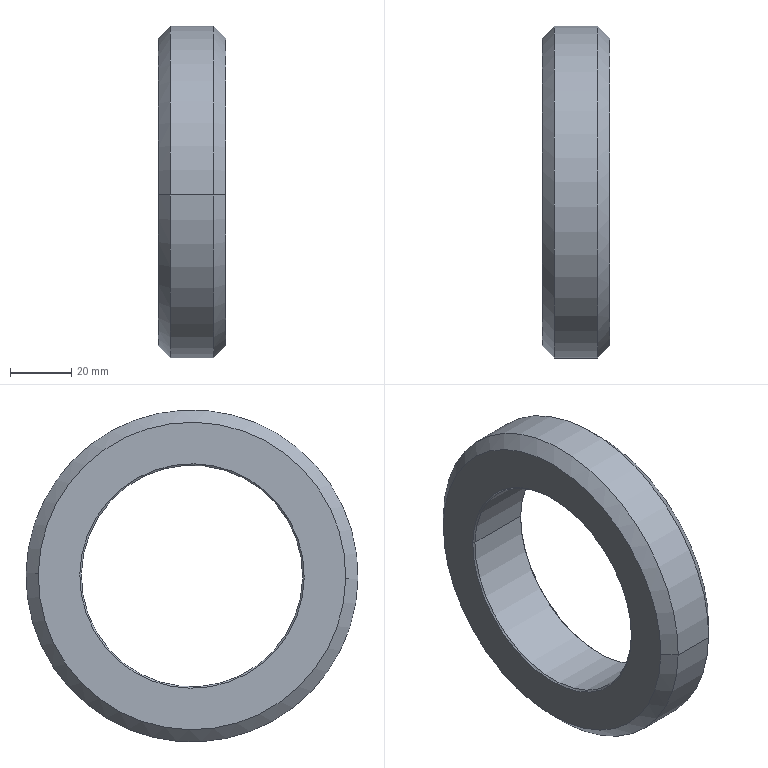Component | SolidWorks | 216InnerTubeAssembly-1_HangingRing-1 | 1 solid | 14 faces | box 22 x 108 x 108 mm | volume 106615 mm3 | cone 8 | cylinder 4 | plane 2 | commonest cylinder face diameters 108 x2 72 x2 | material Alloy Steel
build123d program:
from build123d import *


with BuildPart() as part:
    # Model → Revolve1 (revolve)
    with BuildSketch(Plane.XY):
        Polygon((-0.3448, 49.996), (-0.3448, 36.496), (-0.8448, 35.996), (-21.845, 35.996), (-22.345, 36.496), (-22.345, 49.996), (-18.345, 53.996), (-4.345, 53.996), align=None)
    revolve(axis=Axis((-0.1895, -0.00351, 0), (-1, 0, 0)))


solid = part.part

# Placed as in the assembly
solid = solid.moved(Location((650.924, 0.00351, 0), (0, 0, 0)))
STEP:
#1=CARTESIAN_POINT('',(24.905,2.126,0.03817));
#2=VERTEX_POINT('',#1);
#3=CARTESIAN_POINT('',(24.905,-2.126,-0.03817));
#4=VERTEX_POINT('',#3);
#5=CARTESIAN_POINT('',(24.905,-0.,0.));
#6=DIRECTION('',(1.,0.,0.));
#7=DIRECTION('',(0.,0.9998,0.01796));
#8=AXIS2_PLACEMENT_3D('',#5,#6,#7);
#9=CIRCLE('',#8,2.126);
#10=EDGE_CURVE('',#2,#4,#9,.T.);
#11=ORIENTED_EDGE('',*,*,#10,.T.);
#12=CARTESIAN_POINT('',(25.456,-2.126,-0.03817));
#13=VERTEX_POINT('',#12);
#14=CARTESIAN_POINT('',(25.619,-2.126,-0.03817));
#15=DIRECTION('',(1.,0.,0.));
#16=VECTOR('',#15,39.37);
#17=LINE('',#14,#16);
#18=EDGE_CURVE('',#4,#13,#17,.T.);
#19=ORIENTED_EDGE('',*,*,#18,.T.);
#20=CARTESIAN_POINT('',(25.456,2.126,0.03817));
#21=VERTEX_POINT('',#20);
#22=CARTESIAN_POINT('',(25.456,-0.,0.));
#23=DIRECTION('',(1.,0.,0.));
#24=DIRECTION('',(0.,0.9998,0.01796));
#25=AXIS2_PLACEMENT_3D('',#22,#23,#24);
#26=CIRCLE('',#25,2.126);
#27=EDGE_CURVE('',#21,#13,#26,.T.);
#28=ORIENTED_EDGE('',*,*,#27,.F.);
#29=CARTESIAN_POINT('',(25.619,2.126,0.03817));
#30=DIRECTION('',(1.,0.,0.));
#31=VECTOR('',#30,39.37);
#32=LINE('',#29,#31);
#33=EDGE_CURVE('',#2,#21,#32,.T.);
#34=ORIENTED_EDGE('',*,*,#33,.F.);
#35=EDGE_LOOP('',(#11,#19,#28,#34));
#36=FACE_OUTER_BOUND('',#35,.T.);
#37=CARTESIAN_POINT('',(25.619,-0.,0.));
#38=DIRECTION('',(1.,0.,0.));
#39=DIRECTION('',(0.,0.9998,0.01796));
#40=AXIS2_PLACEMENT_3D('',#37,#38,#39);
#41=CYLINDRICAL_SURFACE('',#40,2.126);
#42=ADVANCED_FACE('',(#36),#41,.T.);
#43=CARTESIAN_POINT('',(24.747,1.968,0.03535));
#44=VERTEX_POINT('',#43);
#45=CARTESIAN_POINT('',(24.747,-1.968,-0.03535));
#46=VERTEX_POINT('',#45);
#47=CARTESIAN_POINT('',(24.747,-0.,0.));
#48=DIRECTION('',(1.,0.,0.));
#49=DIRECTION('',(0.,0.9998,0.01796));
#50=AXIS2_PLACEMENT_3D('',#47,#48,#49);
#51=CIRCLE('',#50,1.969);
#52=EDGE_CURVE('',#44,#46,#51,.T.);
#53=ORIENTED_EDGE('',*,*,#52,.T.);
#54=CARTESIAN_POINT('',(24.905,-2.126,-0.03817));
#55=DIRECTION('',(0.7071,-0.707,-0.0127));
#56=VECTOR('',#55,39.37);
#57=LINE('',#54,#56);
#58=EDGE_CURVE('',#46,#4,#57,.T.);
#59=ORIENTED_EDGE('',*,*,#58,.T.);
#60=ORIENTED_EDGE('',*,*,#10,.F.);
#61=CARTESIAN_POINT('',(24.905,2.126,0.03817));
#62=DIRECTION('',(0.7071,0.707,0.0127));
#63=VECTOR('',#62,39.37);
#64=LINE('',#61,#63);
#65=EDGE_CURVE('',#44,#2,#64,.T.);
#66=ORIENTED_EDGE('',*,*,#65,.F.);
#67=EDGE_LOOP('',(#53,#59,#60,#66));
#68=FACE_OUTER_BOUND('',#67,.T.);
#69=CARTESIAN_POINT('',(24.905,-0.,0.));
#70=DIRECTION('',(1.,0.,0.));
#71=DIRECTION('',(0.,0.9998,0.01796));
#72=AXIS2_PLACEMENT_3D('',#69,#70,#71);
#73=CONICAL_SURFACE('',#72,2.126,0.7854);
#74=ADVANCED_FACE('',(#68),#73,.T.);
#75=CARTESIAN_POINT('',(24.767,-1.417,-0.02545));
#76=VERTEX_POINT('',#75);
#77=CARTESIAN_POINT('',(24.767,1.417,0.02545));
#78=VERTEX_POINT('',#77);
#79=CARTESIAN_POINT('',(24.767,-0.,0.));
#80=DIRECTION('',(1.,0.,0.));
#81=DIRECTION('',(0.,0.9998,0.01796));
#82=AXIS2_PLACEMENT_3D('',#79,#80,#81);
#83=CIRCLE('',#82,1.417);
#84=EDGE_CURVE('',#76,#78,#83,.T.);
#85=ORIENTED_EDGE('',*,*,#84,.T.);
#86=CARTESIAN_POINT('',(24.747,1.437,0.0258));
#87=VERTEX_POINT('',#86);
#88=CARTESIAN_POINT('',(24.747,1.437,0.0258));
#89=DIRECTION('',(-0.7071,0.707,0.0127));
#90=VECTOR('',#89,39.37);
#91=LINE('',#88,#90);
#92=EDGE_CURVE('',#78,#87,#91,.T.);
#93=ORIENTED_EDGE('',*,*,#92,.T.);
#94=CARTESIAN_POINT('',(24.747,-1.437,-0.0258));
#95=VERTEX_POINT('',#94);
#96=CARTESIAN_POINT('',(24.747,-0.,0.));
#97=DIRECTION('',(1.,0.,0.));
#98=DIRECTION('',(0.,0.9998,0.01796));
#99=AXIS2_PLACEMENT_3D('',#96,#97,#98);
#100=CIRCLE('',#99,1.437);
#101=EDGE_CURVE('',#95,#87,#100,.T.);
#102=ORIENTED_EDGE('',*,*,#101,.F.);
#103=CARTESIAN_POINT('',(24.747,-1.437,-0.0258));
#104=DIRECTION('',(-0.7071,-0.707,-0.0127));
#105=VECTOR('',#104,39.37);
#106=LINE('',#103,#105);
#107=EDGE_CURVE('',#76,#95,#106,.T.);
#108=ORIENTED_EDGE('',*,*,#107,.F.);
#109=EDGE_LOOP('',(#85,#93,#102,#108));
#110=FACE_OUTER_BOUND('',#109,.T.);
#111=CARTESIAN_POINT('',(24.747,-0.,0.));
#112=DIRECTION('',(-1.,-0.,0.));
#113=DIRECTION('',(0.,-0.9998,-0.01796));
#114=AXIS2_PLACEMENT_3D('',#111,#112,#113);
#115=CONICAL_SURFACE('',#114,1.437,0.7854);
#116=ADVANCED_FACE('',(#110),#115,.F.);
#117=ORIENTED_EDGE('',*,*,#84,.F.);
#118=CARTESIAN_POINT('',(25.594,-1.417,-0.02545));
#119=VERTEX_POINT('',#118);
#120=CARTESIAN_POINT('',(25.619,-1.417,-0.02545));
#121=DIRECTION('',(1.,0.,0.));
#122=VECTOR('',#121,39.37);
#123=LINE('',#120,#122);
#124=EDGE_CURVE('',#76,#119,#123,.T.);
#125=ORIENTED_EDGE('',*,*,#124,.T.);
#126=CARTESIAN_POINT('',(25.594,1.417,0.02545));
#127=VERTEX_POINT('',#126);
#128=CARTESIAN_POINT('',(25.594,-0.,0.));
#129=DIRECTION('',(1.,0.,0.));
#130=DIRECTION('',(0.,0.9998,0.01796));
#131=AXIS2_PLACEMENT_3D('',#128,#129,#130);
#132=CIRCLE('',#131,1.417);
#133=EDGE_CURVE('',#119,#127,#132,.T.);
#134=ORIENTED_EDGE('',*,*,#133,.T.);
#135=CARTESIAN_POINT('',(25.619,1.417,0.02545));
#136=DIRECTION('',(1.,0.,0.));
#137=VECTOR('',#136,39.37);
#138=LINE('',#135,#137);
#139=EDGE_CURVE('',#78,#127,#138,.T.);
#140=ORIENTED_EDGE('',*,*,#139,.F.);
#141=EDGE_LOOP('',(#117,#125,#134,#140));
#142=FACE_OUTER_BOUND('',#141,.T.);
#143=CARTESIAN_POINT('',(25.619,-0.,0.));
#144=DIRECTION('',(1.,0.,0.));
#145=DIRECTION('',(0.,0.9998,0.01796));
#146=AXIS2_PLACEMENT_3D('',#143,#144,#145);
#147=CYLINDRICAL_SURFACE('',#146,1.417);
#148=ADVANCED_FACE('',(#142),#147,.F.);
#149=ORIENTED_EDGE('',*,*,#133,.F.);
#150=CARTESIAN_POINT('',(25.613,-1.437,-0.0258));
#151=VERTEX_POINT('',#150);
#152=CARTESIAN_POINT('',(25.594,-1.417,-0.02545));
#153=DIRECTION('',(0.7071,-0.707,-0.0127));
#154=VECTOR('',#153,39.37);
#155=LINE('',#152,#154);
#156=EDGE_CURVE('',#119,#151,#155,.T.);
#157=ORIENTED_EDGE('',*,*,#156,.T.);
#158=CARTESIAN_POINT('',(25.613,1.437,0.0258));
#159=VERTEX_POINT('',#158);
#160=CARTESIAN_POINT('',(25.613,-0.,0.));
#161=DIRECTION('',(1.,0.,0.));
#162=DIRECTION('',(0.,0.9998,0.01796));
#163=AXIS2_PLACEMENT_3D('',#160,#161,#162);
#164=CIRCLE('',#163,1.437);
#165=EDGE_CURVE('',#151,#159,#164,.T.);
#166=ORIENTED_EDGE('',*,*,#165,.T.);
#167=CARTESIAN_POINT('',(25.594,1.417,0.02545));
#168=DIRECTION('',(0.7071,0.707,0.0127));
#169=VECTOR('',#168,39.37);
#170=LINE('',#167,#169);
#171=EDGE_CURVE('',#127,#159,#170,.T.);
#172=ORIENTED_EDGE('',*,*,#171,.F.);
#173=EDGE_LOOP('',(#149,#157,#166,#172));
#174=FACE_OUTER_BOUND('',#173,.T.);
#175=CARTESIAN_POINT('',(25.594,-0.,0.));
#176=DIRECTION('',(1.,0.,0.));
#177=DIRECTION('',(0.,0.9998,0.01796));
#178=AXIS2_PLACEMENT_3D('',#175,#176,#177);
#179=CONICAL_SURFACE('',#178,1.417,0.7854);
#180=ADVANCED_FACE('',(#174),#179,.F.);
#181=CARTESIAN_POINT('',(25.613,1.968,0.03535));
#182=VERTEX_POINT('',#181);
#183=CARTESIAN_POINT('',(25.613,-1.968,-0.03535));
#184=VERTEX_POINT('',#183);
#185=CARTESIAN_POINT('',(25.613,-0.,0.));
#186=DIRECTION('',(1.,0.,0.));
#187=DIRECTION('',(0.,0.9998,0.01796));
#188=AXIS2_PLACEMENT_3D('',#185,#186,#187);
#189=CIRCLE('',#188,1.969);
#190=EDGE_CURVE('',#182,#184,#189,.T.);
#191=ORIENTED_EDGE('',*,*,#190,.F.);
#192=CARTESIAN_POINT('',(25.613,1.968,0.03535));
#193=DIRECTION('',(-0.7071,0.707,0.0127));
#194=VECTOR('',#193,39.37);
#195=LINE('',#192,#194);
#196=EDGE_CURVE('',#182,#21,#195,.T.);
#197=ORIENTED_EDGE('',*,*,#196,.T.);
#198=ORIENTED_EDGE('',*,*,#27,.T.);
#199=CARTESIAN_POINT('',(25.613,-1.968,-0.03535));
#200=DIRECTION('',(-0.7071,-0.707,-0.0127));
#201=VECTOR('',#200,39.37);
#202=LINE('',#199,#201);
#203=EDGE_CURVE('',#184,#13,#202,.T.);
#204=ORIENTED_EDGE('',*,*,#203,.F.);
#205=EDGE_LOOP('',(#191,#197,#198,#204));
#206=FACE_OUTER_BOUND('',#205,.T.);
#207=CARTESIAN_POINT('',(25.613,-0.,0.));
#208=DIRECTION('',(-1.,-0.,0.));
#209=DIRECTION('',(0.,-0.9998,-0.01796));
#210=AXIS2_PLACEMENT_3D('',#207,#208,#209);
#211=CONICAL_SURFACE('',#210,1.969,0.7854);
#212=ADVANCED_FACE('',(#206),#211,.T.);
#213=ORIENTED_EDGE('',*,*,#196,.F.);
#214=CARTESIAN_POINT('',(25.613,-0.,0.));
#215=DIRECTION('',(1.,0.,0.));
#216=DIRECTION('',(0.,0.9998,0.01796));
#217=AXIS2_PLACEMENT_3D('',#214,#215,#216);
#218=CIRCLE('',#217,1.969);
#219=EDGE_CURVE('',#184,#182,#218,.T.);
#220=ORIENTED_EDGE('',*,*,#219,.F.);
#221=ORIENTED_EDGE('',*,*,#203,.T.);
#222=CARTESIAN_POINT('',(25.456,-0.,0.));
#223=DIRECTION('',(1.,0.,0.));
#224=DIRECTION('',(0.,0.9998,0.01796));
#225=AXIS2_PLACEMENT_3D('',#222,#223,#224);
#226=CIRCLE('',#225,2.126);
#227=EDGE_CURVE('',#13,#21,#226,.T.);
#228=ORIENTED_EDGE('',*,*,#227,.T.);
#229=EDGE_LOOP('',(#213,#220,#221,#228));
#230=FACE_OUTER_BOUND('',#229,.T.);
#231=CARTESIAN_POINT('',(25.613,-0.,0.));
#232=DIRECTION('',(-1.,-0.,0.));
#233=DIRECTION('',(0.,-0.9998,-0.01796));
#234=AXIS2_PLACEMENT_3D('',#231,#232,#233);
#235=CONICAL_SURFACE('',#234,1.969,0.7854);
#236=ADVANCED_FACE('',(#230),#235,.T.);
#237=ORIENTED_EDGE('',*,*,#219,.T.);
#238=ORIENTED_EDGE('',*,*,#190,.T.);
#239=EDGE_LOOP('',(#237,#238));
#240=FACE_OUTER_BOUND('',#239,.T.);
#241=CARTESIAN_POINT('',(25.613,-0.,0.));
#242=DIRECTION('',(1.,0.,0.));
#243=DIRECTION('',(0.,0.9998,0.01796));
#244=AXIS2_PLACEMENT_3D('',#241,#242,#243);
#245=CIRCLE('',#244,1.437);
#246=EDGE_CURVE('',#159,#151,#245,.T.);
#247=ORIENTED_EDGE('',*,*,#246,.F.);
#248=ORIENTED_EDGE('',*,*,#165,.F.);
#249=EDGE_LOOP('',(#247,#248));
#250=FACE_BOUND('',#249,.T.);
#251=CARTESIAN_POINT('',(25.613,1.968,0.03535));
#252=DIRECTION('',(1.,0.,-0.));
#253=DIRECTION('',(-0.,0.9998,0.01796));
#254=AXIS2_PLACEMENT_3D('',#251,#252,#253);
#255=PLANE('',#254);
#256=ADVANCED_FACE('',(#240,#250),#255,.T.);
#257=ORIENTED_EDGE('',*,*,#156,.F.);
#258=CARTESIAN_POINT('',(25.594,-0.,0.));
#259=DIRECTION('',(1.,0.,0.));
#260=DIRECTION('',(0.,0.9998,0.01796));
#261=AXIS2_PLACEMENT_3D('',#258,#259,#260);
#262=CIRCLE('',#261,1.417);
#263=EDGE_CURVE('',#127,#119,#262,.T.);
#264=ORIENTED_EDGE('',*,*,#263,.F.);
#265=ORIENTED_EDGE('',*,*,#171,.T.);
#266=ORIENTED_EDGE('',*,*,#246,.T.);
#267=EDGE_LOOP('',(#257,#264,#265,#266));
#268=FACE_OUTER_BOUND('',#267,.T.);
#269=CARTESIAN_POINT('',(25.594,-0.,0.));
#270=DIRECTION('',(1.,0.,0.));
#271=DIRECTION('',(0.,0.9998,0.01796));
#272=AXIS2_PLACEMENT_3D('',#269,#270,#271);
#273=CONICAL_SURFACE('',#272,1.417,0.7854);
#274=ADVANCED_FACE('',(#268),#273,.F.);
#275=ORIENTED_EDGE('',*,*,#124,.F.);
#276=CARTESIAN_POINT('',(24.767,-0.,0.));
#277=DIRECTION('',(1.,0.,0.));
#278=DIRECTION('',(0.,0.9998,0.01796));
#279=AXIS2_PLACEMENT_3D('',#276,#277,#278);
#280=CIRCLE('',#279,1.417);
#281=EDGE_CURVE('',#78,#76,#280,.T.);
#282=ORIENTED_EDGE('',*,*,#281,.F.);
#283=ORIENTED_EDGE('',*,*,#139,.T.);
#284=ORIENTED_EDGE('',*,*,#263,.T.);
#285=EDGE_LOOP('',(#275,#282,#283,#284));
#286=FACE_OUTER_BOUND('',#285,.T.);
#287=CARTESIAN_POINT('',(25.619,-0.,0.));
#288=DIRECTION('',(1.,0.,0.));
#289=DIRECTION('',(0.,0.9998,0.01796));
#290=AXIS2_PLACEMENT_3D('',#287,#288,#289);
#291=CYLINDRICAL_SURFACE('',#290,1.417);
#292=ADVANCED_FACE('',(#286),#291,.F.);
#293=ORIENTED_EDGE('',*,*,#92,.F.);
#294=ORIENTED_EDGE('',*,*,#281,.T.);
#295=ORIENTED_EDGE('',*,*,#107,.T.);
#296=CARTESIAN_POINT('',(24.747,-0.,0.));
#297=DIRECTION('',(1.,0.,0.));
#298=DIRECTION('',(0.,0.9998,0.01796));
#299=AXIS2_PLACEMENT_3D('',#296,#297,#298);
#300=CIRCLE('',#299,1.437);
#301=EDGE_CURVE('',#87,#95,#300,.T.);
#302=ORIENTED_EDGE('',*,*,#301,.F.);
#303=EDGE_LOOP('',(#293,#294,#295,#302));
#304=FACE_OUTER_BOUND('',#303,.T.);
#305=CARTESIAN_POINT('',(24.747,-0.,0.));
#306=DIRECTION('',(-1.,-0.,0.));
#307=DIRECTION('',(0.,-0.9998,-0.01796));
#308=AXIS2_PLACEMENT_3D('',#305,#306,#307);
#309=CONICAL_SURFACE('',#308,1.437,0.7854);
#310=ADVANCED_FACE('',(#304),#309,.F.);
#311=ORIENTED_EDGE('',*,*,#101,.T.);
#312=ORIENTED_EDGE('',*,*,#301,.T.);
#313=EDGE_LOOP('',(#311,#312));
#314=FACE_BOUND('',#313,.T.);
#315=ORIENTED_EDGE('',*,*,#52,.F.);
#316=CARTESIAN_POINT('',(24.747,-0.,0.));
#317=DIRECTION('',(1.,0.,0.));
#318=DIRECTION('',(0.,0.9998,0.01796));
#319=AXIS2_PLACEMENT_3D('',#316,#317,#318);
#320=CIRCLE('',#319,1.969);
#321=EDGE_CURVE('',#46,#44,#320,.T.);
#322=ORIENTED_EDGE('',*,*,#321,.F.);
#323=EDGE_LOOP('',(#315,#322));
#324=FACE_OUTER_BOUND('',#323,.T.);
#325=CARTESIAN_POINT('',(24.747,1.437,0.0258));
#326=DIRECTION('',(-1.,-0.,0.));
#327=DIRECTION('',(0.,-0.9998,-0.01796));
#328=AXIS2_PLACEMENT_3D('',#325,#326,#327);
#329=PLANE('',#328);
#330=ADVANCED_FACE('',(#314,#324),#329,.T.);
#331=ORIENTED_EDGE('',*,*,#58,.F.);
#332=ORIENTED_EDGE('',*,*,#321,.T.);
#333=ORIENTED_EDGE('',*,*,#65,.T.);
#334=CARTESIAN_POINT('',(24.905,-0.,0.));
#335=DIRECTION('',(1.,0.,0.));
#336=DIRECTION('',(0.,0.9998,0.01796));
#337=AXIS2_PLACEMENT_3D('',#334,#335,#336);
#338=CIRCLE('',#337,2.126);
#339=EDGE_CURVE('',#4,#2,#338,.T.);
#340=ORIENTED_EDGE('',*,*,#339,.F.);
#341=EDGE_LOOP('',(#331,#332,#333,#340));
#342=FACE_OUTER_BOUND('',#341,.T.);
#343=CARTESIAN_POINT('',(24.905,-0.,0.));
#344=DIRECTION('',(1.,0.,0.));
#345=DIRECTION('',(0.,0.9998,0.01796));
#346=AXIS2_PLACEMENT_3D('',#343,#344,#345);
#347=CONICAL_SURFACE('',#346,2.126,0.7854);
#348=ADVANCED_FACE('',(#342),#347,.T.);
#349=ORIENTED_EDGE('',*,*,#18,.F.);
#350=ORIENTED_EDGE('',*,*,#339,.T.);
#351=ORIENTED_EDGE('',*,*,#33,.T.);
#352=ORIENTED_EDGE('',*,*,#227,.F.);
#353=EDGE_LOOP('',(#349,#350,#351,#352));
#354=FACE_OUTER_BOUND('',#353,.T.);
#355=CARTESIAN_POINT('',(25.619,-0.,0.));
#356=DIRECTION('',(1.,0.,0.));
#357=DIRECTION('',(0.,0.9998,0.01796));
#358=AXIS2_PLACEMENT_3D('',#355,#356,#357);
#359=CYLINDRICAL_SURFACE('',#358,2.126);
#360=ADVANCED_FACE('',(#354),#359,.T.);
#361=CLOSED_SHELL('',(#42,#74,#116,#148,#180,#212,#236,#256,#274,#292,#310,#330,#348,#360));
#362=MANIFOLD_SOLID_BREP('',#361);
#363=CARTESIAN_POINT('',(0.,0.,0.));
#364=DIRECTION('',(0.,0.,1.));
#365=DIRECTION('',(1.,0.,0.));
#366=AXIS2_PLACEMENT_3D('',#363,#364,#365);
#367=(LENGTH_UNIT()NAMED_UNIT(*)SI_UNIT($,.METRE.));
#368=LENGTH_MEASURE_WITH_UNIT(LENGTH_MEASURE(0.0254),#367);
#369=DIMENSIONAL_EXPONENTS(1.,0.,0.,0.,0.,0.,0.);
#370=(CONVERSION_BASED_UNIT('',#368)LENGTH_UNIT()NAMED_UNIT(#369));
#371=UNCERTAINTY_MEASURE_WITH_UNIT(LENGTH_MEASURE(0.00001),#370,'','');
#372=(NAMED_UNIT(*)PLANE_ANGLE_UNIT()SI_UNIT($,.RADIAN.));
#373=(NAMED_UNIT(*)SI_UNIT($,.STERADIAN.)SOLID_ANGLE_UNIT());
#374=(GEOMETRIC_REPRESENTATION_CONTEXT(3)GLOBAL_UNCERTAINTY_ASSIGNED_CONTEXT((#371))GLOBAL_UNIT_ASSIGNED_CONTEXT((#370,#372,#373))REPRESENTATION_CONTEXT('',''));
#375=ADVANCED_BREP_SHAPE_REPRESENTATION('',(#362,#366),#374);
#376=COLOUR_RGB('',0.7922,0.8196,0.9333);
#377=FILL_AREA_STYLE_COLOUR('',#376);
#378=FILL_AREA_STYLE('',(#377));
#379=SURFACE_STYLE_FILL_AREA(#378);
#380=SURFACE_SIDE_STYLE('',(#379));
#381=SURFACE_STYLE_USAGE(.BOTH.,#380);
#382=PRESENTATION_STYLE_ASSIGNMENT((#381));
#383=STYLED_ITEM('',(#382),#362);
#384=PRESENTATION_LAYER_ASSIGNMENT('','',(#383));
#385=(LENGTH_UNIT()NAMED_UNIT(*)SI_UNIT($,.METRE.));
#386=LENGTH_MEASURE_WITH_UNIT(LENGTH_MEASURE(0.0254),#385);
#387=DIMENSIONAL_EXPONENTS(1.,0.,0.,0.,0.,0.,0.);
#388=(CONVERSION_BASED_UNIT('',#386)LENGTH_UNIT()NAMED_UNIT(#387));
#389=UNCERTAINTY_MEASURE_WITH_UNIT(LENGTH_MEASURE(0.00001),#388,'','');
#390=(NAMED_UNIT(*)PLANE_ANGLE_UNIT()SI_UNIT($,.RADIAN.));
#391=(NAMED_UNIT(*)SI_UNIT($,.STERADIAN.)SOLID_ANGLE_UNIT());
#392=(GEOMETRIC_REPRESENTATION_CONTEXT(3)GLOBAL_UNCERTAINTY_ASSIGNED_CONTEXT((#389))GLOBAL_UNIT_ASSIGNED_CONTEXT((#388,#390,#391))REPRESENTATION_CONTEXT('',''));
#393=MECHANICAL_DESIGN_GEOMETRIC_PRESENTATION_REPRESENTATION('',(#383),#392);